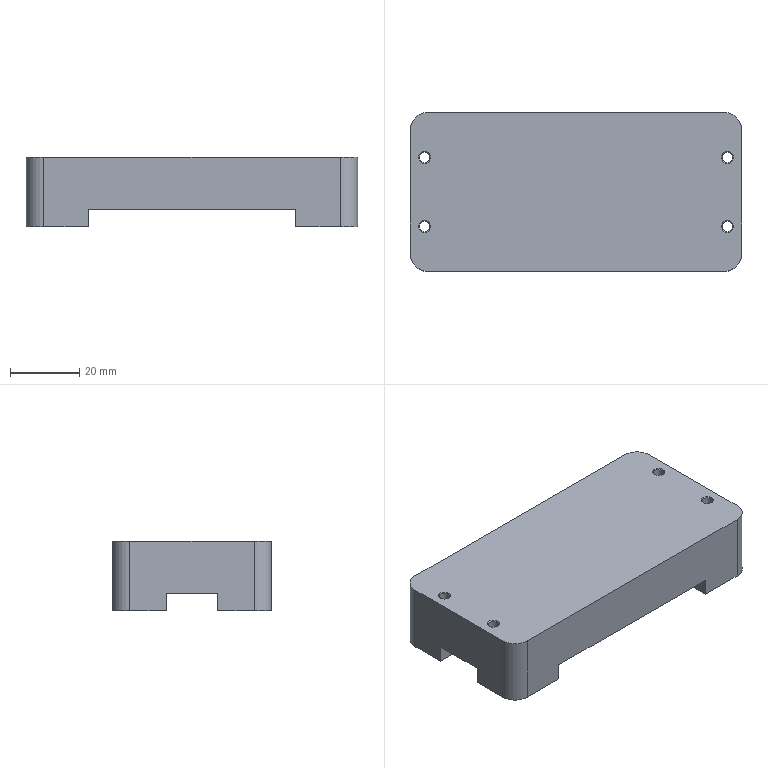Component | NX | BASE_PLATE | 1 solid | 34 faces | volume 70823 mm3 | plane 18 | cylinder 8 | cone 8 | commonest cylinder face diameters 10 x4 3 x4